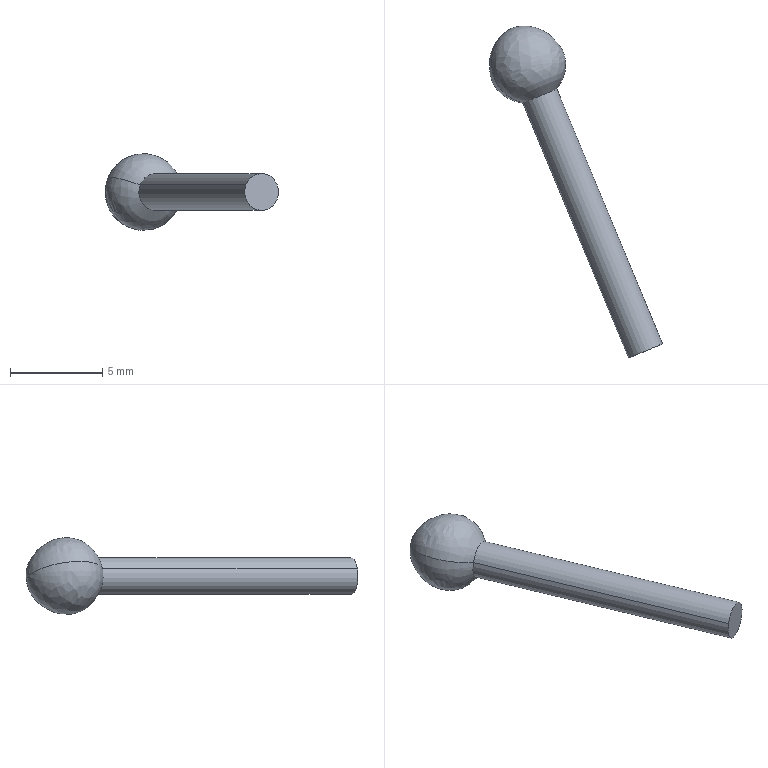Component | SolidWorks | FixedSign-1 | 1 solid | 5 faces | box 9.42 x 18.04 x 4.17 mm | volume 85 mm3 | spline 2 | cylinder 2 | plane 1 | commonest cylinder face diameters 2 x2
build123d program:
from build123d import *

# Parameters (mm, degrees)
SKETCH1_R           = 1
BOSS_EXTRUDE1_DEPTH = 15


with BuildPart() as part:
    # Sketch1 → Boss-Extrude1 (new body)
    with BuildSketch(Plane.XY):
        Circle(SKETCH1_R)
    extrude(amount=BOSS_EXTRUDE1_DEPTH)

    # Sketch2 → Revolve1 (revolve)
    with BuildSketch(Plane(origin=(0, 0, 0), x_dir=(1, 0, 0), z_dir=(0, 1, 0))):
        with BuildLine():
            Line((0, 3.985), (0, 0))
            Line((0, 0), (-1, 0))
            add(Edge.make_bspline(
                [(-1, 0), (-3.105, 1.211), (-1.813, 3.935), (0, 3.985)],
                knots=[0, 0, 0, 0, 1, 1, 1, 1], degree=3))
        make_face()
    revolve(axis=Axis((0, 0, -4.286), (0, 0, 1)))


solid = part.part

# Placed as in the assembly
solid = solid.moved(Location((30.876, 7.06, 430.346), (90, 22.523, -22.52)))
STEP:
#1=COLOUR_RGB('',0.7922,0.8196,0.9333);
#2=FILL_AREA_STYLE_COLOUR('',#1);
#3=FILL_AREA_STYLE('',(#2));
#4=SURFACE_STYLE_FILL_AREA(#3);
#5=SURFACE_SIDE_STYLE('',(#4));
#6=SURFACE_STYLE_USAGE(.BOTH.,#5);
#7=PRESENTATION_STYLE_ASSIGNMENT((#6));
#8=CARTESIAN_POINT('',(1.156,0.4229,16.943));
#9=VERTEX_POINT('',#8);
#10=CARTESIAN_POINT('',(1.182,0.264,16.958));
#11=VERTEX_POINT('',#10);
#12=CARTESIAN_POINT('',(1.156,0.4229,16.943));
#13=CARTESIAN_POINT('',(1.095,0.3958,16.97));
#14=CARTESIAN_POINT('',(1.093,0.2788,16.99));
#15=CARTESIAN_POINT('',(1.182,0.264,16.958));
#16=B_SPLINE_CURVE_WITH_KNOTS('',3,(#12,#13,#14,#15),.UNSPECIFIED.,.F.,.F.,(4,4),(0.,1.),.UNSPECIFIED.);
#17=EDGE_CURVE('',#9,#11,#16,.T.);
#18=ORIENTED_EDGE('',*,*,#17,.F.);
#19=CARTESIAN_POINT('',(1.249,0.2919,16.928));
#20=VERTEX_POINT('',#19);
#21=CARTESIAN_POINT('',(1.156,0.4229,16.943));
#22=CARTESIAN_POINT('',(1.217,0.4464,16.915));
#23=CARTESIAN_POINT('',(1.302,0.3653,16.896));
#24=CARTESIAN_POINT('',(1.249,0.2919,16.928));
#25=B_SPLINE_CURVE_WITH_KNOTS('',3,(#21,#22,#23,#24),.UNSPECIFIED.,.F.,.F.,(4,4),(0.,1.),.UNSPECIFIED.);
#26=EDGE_CURVE('',#9,#20,#25,.T.);
#27=ORIENTED_EDGE('',*,*,#26,.T.);
#28=CARTESIAN_POINT('',(1.216,0.278,16.943));
#29=DIRECTION('',(-0.383,0.9237,0.));
#30=DIRECTION('',(-0.8533,-0.3538,0.383));
#31=AXIS2_PLACEMENT_3D('',#28,#29,#30);
#32=CIRCLE('',#31,0.03937);
#33=EDGE_CURVE('',#20,#11,#32,.T.);
#34=ORIENTED_EDGE('',*,*,#33,.T.);
#35=EDGE_LOOP('',(#18,#27,#34));
#36=FACE_OUTER_BOUND('',#35,.T.);
#37=CARTESIAN_POINT('',(1.156,0.4229,16.943));
#38=CARTESIAN_POINT('',(1.156,0.4229,16.943));
#39=CARTESIAN_POINT('',(1.156,0.4229,16.943));
#40=CARTESIAN_POINT('',(1.156,0.4229,16.943));
#41=CARTESIAN_POINT('',(1.217,0.4464,16.915));
#42=CARTESIAN_POINT('',(1.167,0.4254,16.784));
#43=CARTESIAN_POINT('',(1.045,0.3749,16.838));
#44=CARTESIAN_POINT('',(1.095,0.3958,16.97));
#45=CARTESIAN_POINT('',(1.302,0.3653,16.896));
#46=CARTESIAN_POINT('',(1.215,0.3294,16.67));
#47=CARTESIAN_POINT('',(1.007,0.2429,16.764));
#48=CARTESIAN_POINT('',(1.093,0.2788,16.99));
#49=CARTESIAN_POINT('',(1.249,0.2919,16.928));
#50=CARTESIAN_POINT('',(1.221,0.2803,16.855));
#51=CARTESIAN_POINT('',(1.154,0.2525,16.885));
#52=CARTESIAN_POINT('',(1.182,0.264,16.958));
#53=(BOUNDED_SURFACE()B_SPLINE_SURFACE(3,3,((#37,#38,#39,#40),(#41,#42,#43,#44),(#45,#46,#47,#48),(#49,#50,#51,#52)),.UNSPECIFIED.,.F.,.F.,.T.)B_SPLINE_SURFACE_WITH_KNOTS((4,4),(4,4),(0.,1.),(0.,1.),.UNSPECIFIED.)GEOMETRIC_REPRESENTATION_ITEM()RATIONAL_B_SPLINE_SURFACE(((1.,0.3333,0.3333,1.),(1.,0.3333,0.3333,1.),(1.,0.3333,0.3333,1.),(1.,0.3333,0.3333,1.)))REPRESENTATION_ITEM('')SURFACE());
#54=ADVANCED_FACE('',(#36),#53,.T.);
#55=CARTESIAN_POINT('',(1.475,-0.2536,16.928));
#56=VERTEX_POINT('',#55);
#57=CARTESIAN_POINT('',(1.408,-0.2815,16.958));
#58=VERTEX_POINT('',#57);
#59=CARTESIAN_POINT('',(1.442,-0.2675,16.943));
#60=DIRECTION('',(0.383,-0.9237,0.));
#61=DIRECTION('',(0.8533,0.3538,-0.383));
#62=AXIS2_PLACEMENT_3D('',#59,#60,#61);
#63=CIRCLE('',#62,0.03937);
#64=EDGE_CURVE('',#56,#58,#63,.T.);
#65=ORIENTED_EDGE('',*,*,#64,.F.);
#66=CARTESIAN_POINT('',(1.475,-0.2536,16.928));
#67=DIRECTION('',(-0.383,0.9237,0.));
#68=VECTOR('',#67,39.37);
#69=LINE('',#66,#68);
#70=EDGE_CURVE('',#56,#20,#69,.T.);
#71=ORIENTED_EDGE('',*,*,#70,.T.);
#72=CARTESIAN_POINT('',(1.216,0.278,16.943));
#73=DIRECTION('',(-0.383,0.9237,0.));
#74=DIRECTION('',(-0.8533,-0.3538,0.383));
#75=AXIS2_PLACEMENT_3D('',#72,#73,#74);
#76=CIRCLE('',#75,0.03937);
#77=EDGE_CURVE('',#11,#20,#76,.T.);
#78=ORIENTED_EDGE('',*,*,#77,.F.);
#79=CARTESIAN_POINT('',(1.408,-0.2815,16.958));
#80=DIRECTION('',(-0.383,0.9237,0.));
#81=VECTOR('',#80,39.37);
#82=LINE('',#79,#81);
#83=EDGE_CURVE('',#58,#11,#82,.T.);
#84=ORIENTED_EDGE('',*,*,#83,.F.);
#85=EDGE_LOOP('',(#65,#71,#78,#84));
#86=FACE_OUTER_BOUND('',#85,.T.);
#87=CARTESIAN_POINT('',(1.442,-0.2675,16.943));
#88=DIRECTION('',(-0.383,0.9237,0.));
#89=DIRECTION('',(-0.8533,-0.3538,0.383));
#90=AXIS2_PLACEMENT_3D('',#87,#88,#89);
#91=CYLINDRICAL_SURFACE('',#90,0.03937);
#92=ADVANCED_FACE('',(#86),#91,.T.);
#93=ORIENTED_EDGE('',*,*,#70,.F.);
#94=CARTESIAN_POINT('',(1.442,-0.2675,16.943));
#95=DIRECTION('',(0.383,-0.9237,0.));
#96=DIRECTION('',(0.8533,0.3538,-0.383));
#97=AXIS2_PLACEMENT_3D('',#94,#95,#96);
#98=CIRCLE('',#97,0.03937);
#99=EDGE_CURVE('',#58,#56,#98,.T.);
#100=ORIENTED_EDGE('',*,*,#99,.F.);
#101=ORIENTED_EDGE('',*,*,#83,.T.);
#102=ORIENTED_EDGE('',*,*,#33,.F.);
#103=EDGE_LOOP('',(#93,#100,#101,#102));
#104=FACE_OUTER_BOUND('',#103,.T.);
#105=CARTESIAN_POINT('',(1.442,-0.2675,16.943));
#106=DIRECTION('',(-0.383,0.9237,0.));
#107=DIRECTION('',(-0.8533,-0.3538,0.383));
#108=AXIS2_PLACEMENT_3D('',#105,#106,#107);
#109=CYLINDRICAL_SURFACE('',#108,0.03937);
#110=ADVANCED_FACE('',(#104),#109,.T.);
#111=ORIENTED_EDGE('',*,*,#99,.T.);
#112=ORIENTED_EDGE('',*,*,#64,.T.);
#113=EDGE_LOOP('',(#111,#112));
#114=FACE_OUTER_BOUND('',#113,.T.);
#115=CARTESIAN_POINT('',(1.442,-0.2675,16.943));
#116=DIRECTION('',(0.383,-0.9237,-0.));
#117=DIRECTION('',(0.8533,0.3538,-0.383));
#118=AXIS2_PLACEMENT_3D('',#115,#116,#117);
#119=PLANE('',#118);
#120=ADVANCED_FACE('',(#114),#119,.T.);
#121=ORIENTED_EDGE('',*,*,#26,.F.);
#122=ORIENTED_EDGE('',*,*,#17,.T.);
#123=ORIENTED_EDGE('',*,*,#77,.T.);
#124=EDGE_LOOP('',(#121,#122,#123));
#125=FACE_OUTER_BOUND('',#124,.T.);
#126=CARTESIAN_POINT('',(1.156,0.4229,16.943));
#127=CARTESIAN_POINT('',(1.156,0.4229,16.943));
#128=CARTESIAN_POINT('',(1.156,0.4229,16.943));
#129=CARTESIAN_POINT('',(1.156,0.4229,16.943));
#130=CARTESIAN_POINT('',(1.095,0.3958,16.97));
#131=CARTESIAN_POINT('',(1.146,0.4168,17.102));
#132=CARTESIAN_POINT('',(1.268,0.4673,17.047));
#133=CARTESIAN_POINT('',(1.217,0.4464,16.915));
#134=CARTESIAN_POINT('',(1.093,0.2788,16.99));
#135=CARTESIAN_POINT('',(1.18,0.3146,17.215));
#136=CARTESIAN_POINT('',(1.388,0.4011,17.122));
#137=CARTESIAN_POINT('',(1.302,0.3653,16.896));
#138=CARTESIAN_POINT('',(1.182,0.264,16.958));
#139=CARTESIAN_POINT('',(1.21,0.2756,17.031));
#140=CARTESIAN_POINT('',(1.277,0.3035,17.));
#141=CARTESIAN_POINT('',(1.249,0.2919,16.928));
#142=(BOUNDED_SURFACE()B_SPLINE_SURFACE(3,3,((#126,#127,#128,#129),(#130,#131,#132,#133),(#134,#135,#136,#137),(#138,#139,#140,#141)),.UNSPECIFIED.,.F.,.F.,.T.)B_SPLINE_SURFACE_WITH_KNOTS((4,4),(4,4),(0.,1.),(0.,1.),.UNSPECIFIED.)GEOMETRIC_REPRESENTATION_ITEM()RATIONAL_B_SPLINE_SURFACE(((1.,0.3333,0.3333,1.),(1.,0.3333,0.3333,1.),(1.,0.3333,0.3333,1.),(1.,0.3333,0.3333,1.)))REPRESENTATION_ITEM('')SURFACE());
#143=ADVANCED_FACE('',(#125),#142,.T.);
#144=CLOSED_SHELL('',(#54,#92,#110,#120,#143));
#145=MANIFOLD_SOLID_BREP('',#144);
#146=STYLED_ITEM('',(#7),#145);
#147=(LENGTH_UNIT()NAMED_UNIT(*)SI_UNIT($,.METRE.));
#148=LENGTH_MEASURE_WITH_UNIT(LENGTH_MEASURE(0.0254),#147);
#149=DIMENSIONAL_EXPONENTS(1.,0.,0.,0.,0.,0.,0.);
#150=(CONVERSION_BASED_UNIT('',#148)LENGTH_UNIT()NAMED_UNIT(#149));
#151=UNCERTAINTY_MEASURE_WITH_UNIT(LENGTH_MEASURE(0.00001),#150,'','');
#152=(NAMED_UNIT(*)PLANE_ANGLE_UNIT()SI_UNIT($,.RADIAN.));
#153=(NAMED_UNIT(*)SI_UNIT($,.STERADIAN.)SOLID_ANGLE_UNIT());
#154=(GEOMETRIC_REPRESENTATION_CONTEXT(3)GLOBAL_UNCERTAINTY_ASSIGNED_CONTEXT((#151))GLOBAL_UNIT_ASSIGNED_CONTEXT((#150,#152,#153))REPRESENTATION_CONTEXT('',''));
#155=MECHANICAL_DESIGN_GEOMETRIC_PRESENTATION_REPRESENTATION('',(#146),#154);
#156=CARTESIAN_POINT('',(0.,0.,0.));
#157=DIRECTION('',(0.,0.,1.));
#158=DIRECTION('',(1.,0.,0.));
#159=AXIS2_PLACEMENT_3D('',#156,#157,#158);
#160=(LENGTH_UNIT()NAMED_UNIT(*)SI_UNIT($,.METRE.));
#161=LENGTH_MEASURE_WITH_UNIT(LENGTH_MEASURE(0.0254),#160);
#162=DIMENSIONAL_EXPONENTS(1.,0.,0.,0.,0.,0.,0.);
#163=(CONVERSION_BASED_UNIT('',#161)LENGTH_UNIT()NAMED_UNIT(#162));
#164=UNCERTAINTY_MEASURE_WITH_UNIT(LENGTH_MEASURE(0.00001),#163,'','');
#165=(NAMED_UNIT(*)PLANE_ANGLE_UNIT()SI_UNIT($,.RADIAN.));
#166=(NAMED_UNIT(*)SI_UNIT($,.STERADIAN.)SOLID_ANGLE_UNIT());
#167=(GEOMETRIC_REPRESENTATION_CONTEXT(3)GLOBAL_UNCERTAINTY_ASSIGNED_CONTEXT((#164))GLOBAL_UNIT_ASSIGNED_CONTEXT((#163,#165,#166))REPRESENTATION_CONTEXT('',''));
#168=ADVANCED_BREP_SHAPE_REPRESENTATION('',(#145,#159),#167);
#169=PRESENTATION_LAYER_ASSIGNMENT('','',(#146));